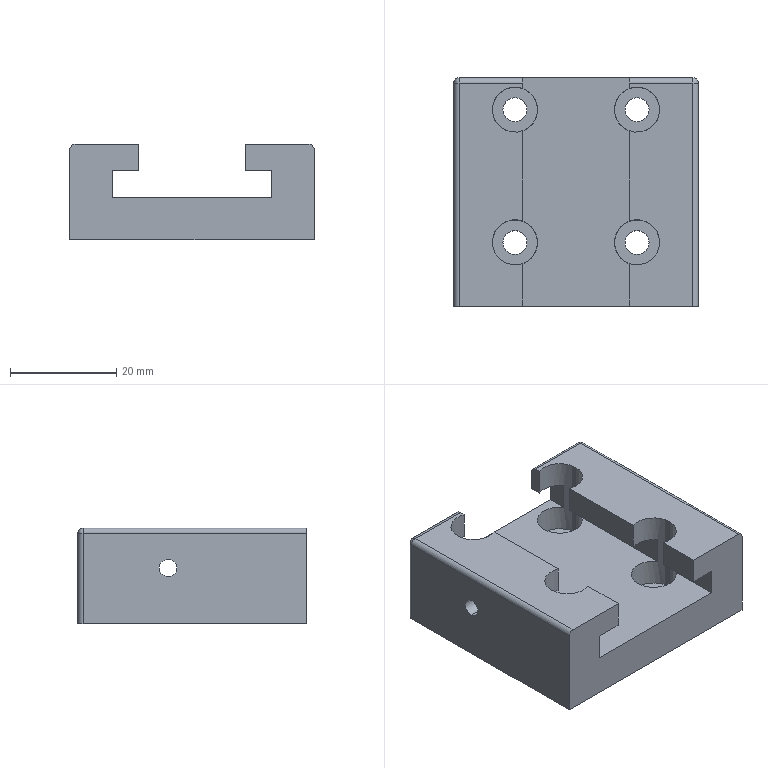Component | SolidWorks | 18ZTJ-NVT-01-009-1 | 1 solid | 983 faces | box 46 x 43 x 18 mm | volume 22282 mm3 | plane 807 | spline 140 | cylinder 30 | cone 4 | sphere 2 | commonest cylinder face diameters 3.3 x8 8.5 x8 4.5 x8 2 x6 | material #45